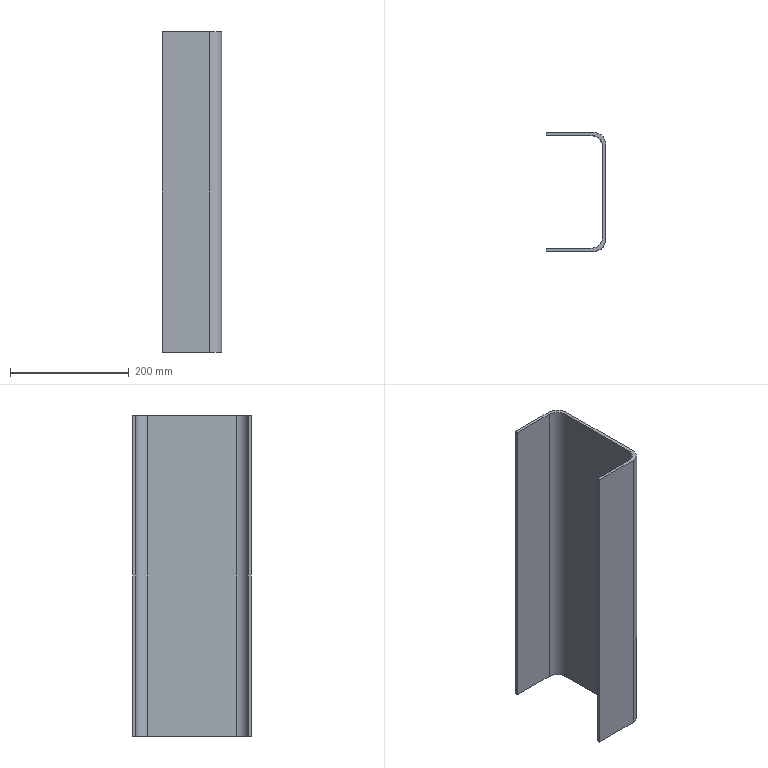Component | NX | PERFIL_U | 1 solid | 14 faces | box 100 x 200 x 540 mm | volume 1053000 mm3 | plane 10 | cylinder 4 | commonest cylinder face diameters 40 x4
STEP:
#1=CARTESIAN_POINT('',(0.,0.,0.));
#2=DIRECTION('',(0.,0.,1.));
#3=DIRECTION('',(1.,0.,0.));
#4=AXIS2_PLACEMENT_3D('',#1,#2,#3);
#5=CARTESIAN_POINT('',(0.,-234.8,700.));
#6=VERTEX_POINT('',#5);
#7=CARTESIAN_POINT('',(80.,-234.8,700.));
#8=VERTEX_POINT('',#7);
#9=CARTESIAN_POINT('',(0.,-234.8,700.));
#10=DIRECTION('',(1.,0.,0.));
#11=VECTOR('',#10,1.);
#12=LINE('',#9,#11);
#13=CARTESIAN_POINT('',(0.,-234.8,160.));
#14=DIRECTION('',(0.,-1.,0.));
#15=DIRECTION('',(1.,0.,0.));
#16=AXIS2_PLACEMENT_3D('',#13,#14,#15);
#17=PLANE('',#16);
#18=CARTESIAN_POINT('',(0.,540.));
#19=DIRECTION('',(1.,0.));
#20=VECTOR('',#19,1.);
#21=LINE('',#18,#20);
#22=(GEOMETRIC_REPRESENTATION_CONTEXT(2)PARAMETRIC_REPRESENTATION_CONTEXT()REPRESENTATION_CONTEXT('',''));
#23=DEFINITIONAL_REPRESENTATION('',(#21),#22);
#24=PCURVE('',#17,#23);
#25=CARTESIAN_POINT('',(100.,-234.8,700.));
#26=DIRECTION('',(0.,0.,-1.));
#27=DIRECTION('',(1.,0.,0.));
#28=AXIS2_PLACEMENT_3D('',#25,#26,#27);
#29=PLANE('',#28);
#30=CARTESIAN_POINT('',(-100.,0.));
#31=DIRECTION('',(1.,0.));
#32=VECTOR('',#31,1.);
#33=LINE('',#30,#32);
#34=(GEOMETRIC_REPRESENTATION_CONTEXT(2)PARAMETRIC_REPRESENTATION_CONTEXT()REPRESENTATION_CONTEXT('',''));
#35=DEFINITIONAL_REPRESENTATION('',(#33),#34);
#36=PCURVE('',#29,#35);
#37=SURFACE_CURVE('',#12,(#24,#36),.PCURVE_S1.);
#38=EDGE_CURVE('',#6,#8,#37,.T.);
#39=ORIENTED_EDGE('',*,*,#38,.T.);
#40=CARTESIAN_POINT('',(80.,-234.8,160.));
#41=VERTEX_POINT('',#40);
#42=CARTESIAN_POINT('',(80.,-234.8,160.));
#43=DIRECTION('',(0.,0.,-1.));
#44=VECTOR('',#43,1.);
#45=LINE('',#42,#44);
#46=CARTESIAN_POINT('',(80.,0.));
#47=DIRECTION('',(0.,-1.));
#48=VECTOR('',#47,1.);
#49=LINE('',#46,#48);
#50=(GEOMETRIC_REPRESENTATION_CONTEXT(2)PARAMETRIC_REPRESENTATION_CONTEXT()REPRESENTATION_CONTEXT('',''));
#51=DEFINITIONAL_REPRESENTATION('',(#49),#50);
#52=PCURVE('',#17,#51);
#53=CARTESIAN_POINT('',(80.,-254.8,160.));
#54=DIRECTION('',(0.,0.,1.));
#55=DIRECTION('',(-1.,0.,0.));
#56=AXIS2_PLACEMENT_3D('',#53,#54,#55);
#57=CYLINDRICAL_SURFACE('',#56,20.);
#58=CARTESIAN_POINT('',(4.712,0.));
#59=DIRECTION('',(0.,-1.));
#60=VECTOR('',#59,1.);
#61=LINE('',#58,#60);
#62=(GEOMETRIC_REPRESENTATION_CONTEXT(2)PARAMETRIC_REPRESENTATION_CONTEXT()REPRESENTATION_CONTEXT('',''));
#63=DEFINITIONAL_REPRESENTATION('',(#61),#62);
#64=PCURVE('',#57,#63);
#65=SURFACE_CURVE('',#45,(#52,#64),.PCURVE_S1.);
#66=EDGE_CURVE('',#8,#41,#65,.T.);
#67=ORIENTED_EDGE('',*,*,#66,.T.);
#68=CARTESIAN_POINT('',(0.,-234.8,160.));
#69=VERTEX_POINT('',#68);
#70=CARTESIAN_POINT('',(0.,-234.8,160.));
#71=DIRECTION('',(1.,0.,0.));
#72=VECTOR('',#71,1.);
#73=LINE('',#70,#72);
#74=CARTESIAN_POINT('',(0.,0.));
#75=DIRECTION('',(1.,0.));
#76=VECTOR('',#75,1.);
#77=LINE('',#74,#76);
#78=(GEOMETRIC_REPRESENTATION_CONTEXT(2)PARAMETRIC_REPRESENTATION_CONTEXT()REPRESENTATION_CONTEXT('',''));
#79=DEFINITIONAL_REPRESENTATION('',(#77),#78);
#80=PCURVE('',#17,#79);
#81=CARTESIAN_POINT('',(100.,-234.8,160.));
#82=DIRECTION('',(0.,0.,-1.));
#83=DIRECTION('',(1.,0.,0.));
#84=AXIS2_PLACEMENT_3D('',#81,#82,#83);
#85=PLANE('',#84);
#86=CARTESIAN_POINT('',(-100.,0.));
#87=DIRECTION('',(1.,0.));
#88=VECTOR('',#87,1.);
#89=LINE('',#86,#88);
#90=(GEOMETRIC_REPRESENTATION_CONTEXT(2)PARAMETRIC_REPRESENTATION_CONTEXT()REPRESENTATION_CONTEXT('',''));
#91=DEFINITIONAL_REPRESENTATION('',(#89),#90);
#92=PCURVE('',#85,#91);
#93=SURFACE_CURVE('',#73,(#80,#92),.PCURVE_S1.);
#94=EDGE_CURVE('',#69,#41,#93,.T.);
#95=ORIENTED_EDGE('',*,*,#94,.F.);
#96=CARTESIAN_POINT('',(0.,-234.8,160.));
#97=DIRECTION('',(0.,0.,1.));
#98=VECTOR('',#97,1.);
#99=LINE('',#96,#98);
#100=CARTESIAN_POINT('',(0.,0.));
#101=DIRECTION('',(0.,1.));
#102=VECTOR('',#101,1.);
#103=LINE('',#100,#102);
#104=(GEOMETRIC_REPRESENTATION_CONTEXT(2)PARAMETRIC_REPRESENTATION_CONTEXT()REPRESENTATION_CONTEXT('',''));
#105=DEFINITIONAL_REPRESENTATION('',(#103),#104);
#106=PCURVE('',#17,#105);
#107=CARTESIAN_POINT('',(0.,-239.8,160.));
#108=DIRECTION('',(1.,0.,0.));
#109=DIRECTION('',(0.,1.,0.));
#110=AXIS2_PLACEMENT_3D('',#107,#108,#109);
#111=PLANE('',#110);
#112=CARTESIAN_POINT('',(5.,0.));
#113=DIRECTION('',(0.,1.));
#114=VECTOR('',#113,1.);
#115=LINE('',#112,#114);
#116=(GEOMETRIC_REPRESENTATION_CONTEXT(2)PARAMETRIC_REPRESENTATION_CONTEXT()REPRESENTATION_CONTEXT('',''));
#117=DEFINITIONAL_REPRESENTATION('',(#115),#116);
#118=PCURVE('',#111,#117);
#119=SURFACE_CURVE('',#99,(#106,#118),.PCURVE_S1.);
#120=EDGE_CURVE('',#69,#6,#119,.T.);
#121=ORIENTED_EDGE('',*,*,#120,.T.);
#122=EDGE_LOOP('',(#39,#67,#95,#121));
#123=FACE_BOUND('',#122,.T.);
#124=ADVANCED_FACE('',(#123),#17,.F.);
#125=CARTESIAN_POINT('',(100.,-254.8,700.));
#126=VERTEX_POINT('',#125);
#127=CARTESIAN_POINT('',(100.,-414.8,700.));
#128=VERTEX_POINT('',#127);
#129=CARTESIAN_POINT('',(100.,-234.8,700.));
#130=DIRECTION('',(0.,-1.,0.));
#131=VECTOR('',#130,1.);
#132=LINE('',#129,#131);
#133=CARTESIAN_POINT('',(100.,-234.8,160.));
#134=DIRECTION('',(-1.,0.,0.));
#135=DIRECTION('',(0.,-1.,0.));
#136=AXIS2_PLACEMENT_3D('',#133,#134,#135);
#137=PLANE('',#136);
#138=CARTESIAN_POINT('',(0.,540.));
#139=DIRECTION('',(1.,0.));
#140=VECTOR('',#139,1.);
#141=LINE('',#138,#140);
#142=(GEOMETRIC_REPRESENTATION_CONTEXT(2)PARAMETRIC_REPRESENTATION_CONTEXT()REPRESENTATION_CONTEXT('',''));
#143=DEFINITIONAL_REPRESENTATION('',(#141),#142);
#144=PCURVE('',#137,#143);
#145=CARTESIAN_POINT('',(0.,0.));
#146=DIRECTION('',(0.,1.));
#147=VECTOR('',#146,1.);
#148=LINE('',#145,#147);
#149=(GEOMETRIC_REPRESENTATION_CONTEXT(2)PARAMETRIC_REPRESENTATION_CONTEXT()REPRESENTATION_CONTEXT('',''));
#150=DEFINITIONAL_REPRESENTATION('',(#148),#149);
#151=PCURVE('',#29,#150);
#152=SURFACE_CURVE('',#132,(#144,#151),.PCURVE_S1.);
#153=EDGE_CURVE('',#126,#128,#152,.T.);
#154=ORIENTED_EDGE('',*,*,#153,.T.);
#155=CARTESIAN_POINT('',(100.,-414.8,160.));
#156=VERTEX_POINT('',#155);
#157=CARTESIAN_POINT('',(100.,-414.8,160.));
#158=DIRECTION('',(0.,0.,-1.));
#159=VECTOR('',#158,1.);
#160=LINE('',#157,#159);
#161=CARTESIAN_POINT('',(180.,0.));
#162=DIRECTION('',(0.,-1.));
#163=VECTOR('',#162,1.);
#164=LINE('',#161,#163);
#165=(GEOMETRIC_REPRESENTATION_CONTEXT(2)PARAMETRIC_REPRESENTATION_CONTEXT()REPRESENTATION_CONTEXT('',''));
#166=DEFINITIONAL_REPRESENTATION('',(#164),#165);
#167=PCURVE('',#137,#166);
#168=CARTESIAN_POINT('',(80.,-414.8,160.));
#169=DIRECTION('',(0.,0.,1.));
#170=DIRECTION('',(-1.,0.,0.));
#171=AXIS2_PLACEMENT_3D('',#168,#169,#170);
#172=CYLINDRICAL_SURFACE('',#171,20.);
#173=CARTESIAN_POINT('',(3.142,0.));
#174=DIRECTION('',(0.,-1.));
#175=VECTOR('',#174,1.);
#176=LINE('',#173,#175);
#177=(GEOMETRIC_REPRESENTATION_CONTEXT(2)PARAMETRIC_REPRESENTATION_CONTEXT()REPRESENTATION_CONTEXT('',''));
#178=DEFINITIONAL_REPRESENTATION('',(#176),#177);
#179=PCURVE('',#172,#178);
#180=SURFACE_CURVE('',#160,(#167,#179),.PCURVE_S1.);
#181=EDGE_CURVE('',#128,#156,#180,.T.);
#182=ORIENTED_EDGE('',*,*,#181,.T.);
#183=CARTESIAN_POINT('',(100.,-254.8,160.));
#184=VERTEX_POINT('',#183);
#185=CARTESIAN_POINT('',(100.,-234.8,160.));
#186=DIRECTION('',(0.,-1.,0.));
#187=VECTOR('',#186,1.);
#188=LINE('',#185,#187);
#189=CARTESIAN_POINT('',(0.,0.));
#190=DIRECTION('',(1.,0.));
#191=VECTOR('',#190,1.);
#192=LINE('',#189,#191);
#193=(GEOMETRIC_REPRESENTATION_CONTEXT(2)PARAMETRIC_REPRESENTATION_CONTEXT()REPRESENTATION_CONTEXT('',''));
#194=DEFINITIONAL_REPRESENTATION('',(#192),#193);
#195=PCURVE('',#137,#194);
#196=CARTESIAN_POINT('',(0.,0.));
#197=DIRECTION('',(0.,1.));
#198=VECTOR('',#197,1.);
#199=LINE('',#196,#198);
#200=(GEOMETRIC_REPRESENTATION_CONTEXT(2)PARAMETRIC_REPRESENTATION_CONTEXT()REPRESENTATION_CONTEXT('',''));
#201=DEFINITIONAL_REPRESENTATION('',(#199),#200);
#202=PCURVE('',#85,#201);
#203=SURFACE_CURVE('',#188,(#195,#202),.PCURVE_S1.);
#204=EDGE_CURVE('',#184,#156,#203,.T.);
#205=ORIENTED_EDGE('',*,*,#204,.F.);
#206=CARTESIAN_POINT('',(100.,-254.8,160.));
#207=DIRECTION('',(0.,0.,1.));
#208=VECTOR('',#207,1.);
#209=LINE('',#206,#208);
#210=CARTESIAN_POINT('',(20.,0.));
#211=DIRECTION('',(0.,1.));
#212=VECTOR('',#211,1.);
#213=LINE('',#210,#212);
#214=(GEOMETRIC_REPRESENTATION_CONTEXT(2)PARAMETRIC_REPRESENTATION_CONTEXT()REPRESENTATION_CONTEXT('',''));
#215=DEFINITIONAL_REPRESENTATION('',(#213),#214);
#216=PCURVE('',#137,#215);
#217=CARTESIAN_POINT('',(3.142,0.));
#218=DIRECTION('',(0.,1.));
#219=VECTOR('',#218,1.);
#220=LINE('',#217,#219);
#221=(GEOMETRIC_REPRESENTATION_CONTEXT(2)PARAMETRIC_REPRESENTATION_CONTEXT()REPRESENTATION_CONTEXT('',''));
#222=DEFINITIONAL_REPRESENTATION('',(#220),#221);
#223=PCURVE('',#57,#222);
#224=SURFACE_CURVE('',#209,(#216,#223),.PCURVE_S1.);
#225=EDGE_CURVE('',#184,#126,#224,.T.);
#226=ORIENTED_EDGE('',*,*,#225,.T.);
#227=EDGE_LOOP('',(#154,#182,#205,#226));
#228=FACE_BOUND('',#227,.T.);
#229=ADVANCED_FACE('',(#228),#137,.F.);
#230=CARTESIAN_POINT('',(80.,-434.8,160.));
#231=VERTEX_POINT('',#230);
#232=CARTESIAN_POINT('',(0.,-434.8,160.));
#233=VERTEX_POINT('',#232);
#234=CARTESIAN_POINT('',(100.,-434.8,160.));
#235=DIRECTION('',(-1.,0.,0.));
#236=VECTOR('',#235,1.);
#237=LINE('',#234,#236);
#238=CARTESIAN_POINT('',(100.,-434.8,160.));
#239=DIRECTION('',(0.,1.,0.));
#240=DIRECTION('',(-1.,0.,0.));
#241=AXIS2_PLACEMENT_3D('',#238,#239,#240);
#242=PLANE('',#241);
#243=CARTESIAN_POINT('',(0.,0.));
#244=DIRECTION('',(1.,0.));
#245=VECTOR('',#244,1.);
#246=LINE('',#243,#245);
#247=(GEOMETRIC_REPRESENTATION_CONTEXT(2)PARAMETRIC_REPRESENTATION_CONTEXT()REPRESENTATION_CONTEXT('',''));
#248=DEFINITIONAL_REPRESENTATION('',(#246),#247);
#249=PCURVE('',#242,#248);
#250=CARTESIAN_POINT('',(0.,200.));
#251=DIRECTION('',(-1.,0.));
#252=VECTOR('',#251,1.);
#253=LINE('',#250,#252);
#254=(GEOMETRIC_REPRESENTATION_CONTEXT(2)PARAMETRIC_REPRESENTATION_CONTEXT()REPRESENTATION_CONTEXT('',''));
#255=DEFINITIONAL_REPRESENTATION('',(#253),#254);
#256=PCURVE('',#85,#255);
#257=SURFACE_CURVE('',#237,(#249,#256),.PCURVE_S1.);
#258=EDGE_CURVE('',#231,#233,#257,.T.);
#259=ORIENTED_EDGE('',*,*,#258,.F.);
#260=CARTESIAN_POINT('',(80.,-434.8,700.));
#261=VERTEX_POINT('',#260);
#262=CARTESIAN_POINT('',(80.,-434.8,160.));
#263=DIRECTION('',(0.,0.,1.));
#264=VECTOR('',#263,1.);
#265=LINE('',#262,#264);
#266=CARTESIAN_POINT('',(20.,0.));
#267=DIRECTION('',(0.,1.));
#268=VECTOR('',#267,1.);
#269=LINE('',#266,#268);
#270=(GEOMETRIC_REPRESENTATION_CONTEXT(2)PARAMETRIC_REPRESENTATION_CONTEXT()REPRESENTATION_CONTEXT('',''));
#271=DEFINITIONAL_REPRESENTATION('',(#269),#270);
#272=PCURVE('',#242,#271);
#273=CARTESIAN_POINT('',(1.571,0.));
#274=DIRECTION('',(0.,1.));
#275=VECTOR('',#274,1.);
#276=LINE('',#273,#275);
#277=(GEOMETRIC_REPRESENTATION_CONTEXT(2)PARAMETRIC_REPRESENTATION_CONTEXT()REPRESENTATION_CONTEXT('',''));
#278=DEFINITIONAL_REPRESENTATION('',(#276),#277);
#279=PCURVE('',#172,#278);
#280=SURFACE_CURVE('',#265,(#272,#279),.PCURVE_S1.);
#281=EDGE_CURVE('',#231,#261,#280,.T.);
#282=ORIENTED_EDGE('',*,*,#281,.T.);
#283=CARTESIAN_POINT('',(0.,-434.8,700.));
#284=VERTEX_POINT('',#283);
#285=CARTESIAN_POINT('',(100.,-434.8,700.));
#286=DIRECTION('',(-1.,0.,0.));
#287=VECTOR('',#286,1.);
#288=LINE('',#285,#287);
#289=CARTESIAN_POINT('',(0.,540.));
#290=DIRECTION('',(1.,0.));
#291=VECTOR('',#290,1.);
#292=LINE('',#289,#291);
#293=(GEOMETRIC_REPRESENTATION_CONTEXT(2)PARAMETRIC_REPRESENTATION_CONTEXT()REPRESENTATION_CONTEXT('',''));
#294=DEFINITIONAL_REPRESENTATION('',(#292),#293);
#295=PCURVE('',#242,#294);
#296=CARTESIAN_POINT('',(0.,200.));
#297=DIRECTION('',(-1.,0.));
#298=VECTOR('',#297,1.);
#299=LINE('',#296,#298);
#300=(GEOMETRIC_REPRESENTATION_CONTEXT(2)PARAMETRIC_REPRESENTATION_CONTEXT()REPRESENTATION_CONTEXT('',''));
#301=DEFINITIONAL_REPRESENTATION('',(#299),#300);
#302=PCURVE('',#29,#301);
#303=SURFACE_CURVE('',#288,(#295,#302),.PCURVE_S1.);
#304=EDGE_CURVE('',#261,#284,#303,.T.);
#305=ORIENTED_EDGE('',*,*,#304,.T.);
#306=CARTESIAN_POINT('',(0.,-434.8,160.));
#307=DIRECTION('',(0.,0.,1.));
#308=VECTOR('',#307,1.);
#309=LINE('',#306,#308);
#310=CARTESIAN_POINT('',(100.,0.));
#311=DIRECTION('',(0.,1.));
#312=VECTOR('',#311,1.);
#313=LINE('',#310,#312);
#314=(GEOMETRIC_REPRESENTATION_CONTEXT(2)PARAMETRIC_REPRESENTATION_CONTEXT()REPRESENTATION_CONTEXT('',''));
#315=DEFINITIONAL_REPRESENTATION('',(#313),#314);
#316=PCURVE('',#242,#315);
#317=CARTESIAN_POINT('',(0.,-434.8,160.));
#318=DIRECTION('',(1.,0.,0.));
#319=DIRECTION('',(0.,1.,0.));
#320=AXIS2_PLACEMENT_3D('',#317,#318,#319);
#321=PLANE('',#320);
#322=CARTESIAN_POINT('',(0.,0.));
#323=DIRECTION('',(0.,1.));
#324=VECTOR('',#323,1.);
#325=LINE('',#322,#324);
#326=(GEOMETRIC_REPRESENTATION_CONTEXT(2)PARAMETRIC_REPRESENTATION_CONTEXT()REPRESENTATION_CONTEXT('',''));
#327=DEFINITIONAL_REPRESENTATION('',(#325),#326);
#328=PCURVE('',#321,#327);
#329=SURFACE_CURVE('',#309,(#316,#328),.PCURVE_S1.);
#330=EDGE_CURVE('',#233,#284,#329,.T.);
#331=ORIENTED_EDGE('',*,*,#330,.F.);
#332=EDGE_LOOP('',(#259,#282,#305,#331));
#333=FACE_BOUND('',#332,.T.);
#334=ADVANCED_FACE('',(#333),#242,.F.);
#335=CARTESIAN_POINT('',(0.,-429.8,700.));
#336=VERTEX_POINT('',#335);
#337=CARTESIAN_POINT('',(0.,-434.8,700.));
#338=DIRECTION('',(0.,1.,0.));
#339=VECTOR('',#338,1.);
#340=LINE('',#337,#339);
#341=CARTESIAN_POINT('',(0.,540.));
#342=DIRECTION('',(1.,0.));
#343=VECTOR('',#342,1.);
#344=LINE('',#341,#343);
#345=(GEOMETRIC_REPRESENTATION_CONTEXT(2)PARAMETRIC_REPRESENTATION_CONTEXT()REPRESENTATION_CONTEXT('',''));
#346=DEFINITIONAL_REPRESENTATION('',(#344),#345);
#347=PCURVE('',#321,#346);
#348=CARTESIAN_POINT('',(-100.,200.));
#349=DIRECTION('',(0.,-1.));
#350=VECTOR('',#349,1.);
#351=LINE('',#348,#350);
#352=(GEOMETRIC_REPRESENTATION_CONTEXT(2)PARAMETRIC_REPRESENTATION_CONTEXT()REPRESENTATION_CONTEXT('',''));
#353=DEFINITIONAL_REPRESENTATION('',(#351),#352);
#354=PCURVE('',#29,#353);
#355=SURFACE_CURVE('',#340,(#347,#354),.PCURVE_S1.);
#356=EDGE_CURVE('',#284,#336,#355,.T.);
#357=ORIENTED_EDGE('',*,*,#356,.T.);
#358=CARTESIAN_POINT('',(0.,-429.8,160.));
#359=VERTEX_POINT('',#358);
#360=CARTESIAN_POINT('',(0.,-429.8,160.));
#361=DIRECTION('',(0.,0.,1.));
#362=VECTOR('',#361,1.);
#363=LINE('',#360,#362);
#364=CARTESIAN_POINT('',(5.,0.));
#365=DIRECTION('',(0.,1.));
#366=VECTOR('',#365,1.);
#367=LINE('',#364,#366);
#368=(GEOMETRIC_REPRESENTATION_CONTEXT(2)PARAMETRIC_REPRESENTATION_CONTEXT()REPRESENTATION_CONTEXT('',''));
#369=DEFINITIONAL_REPRESENTATION('',(#367),#368);
#370=PCURVE('',#321,#369);
#371=CARTESIAN_POINT('',(0.,-429.8,160.));
#372=DIRECTION('',(0.,-1.,0.));
#373=DIRECTION('',(1.,0.,0.));
#374=AXIS2_PLACEMENT_3D('',#371,#372,#373);
#375=PLANE('',#374);
#376=CARTESIAN_POINT('',(0.,0.));
#377=DIRECTION('',(0.,1.));
#378=VECTOR('',#377,1.);
#379=LINE('',#376,#378);
#380=(GEOMETRIC_REPRESENTATION_CONTEXT(2)PARAMETRIC_REPRESENTATION_CONTEXT()REPRESENTATION_CONTEXT('',''));
#381=DEFINITIONAL_REPRESENTATION('',(#379),#380);
#382=PCURVE('',#375,#381);
#383=SURFACE_CURVE('',#363,(#370,#382),.PCURVE_S1.);
#384=EDGE_CURVE('',#359,#336,#383,.T.);
#385=ORIENTED_EDGE('',*,*,#384,.F.);
#386=CARTESIAN_POINT('',(0.,-434.8,160.));
#387=DIRECTION('',(0.,1.,0.));
#388=VECTOR('',#387,1.);
#389=LINE('',#386,#388);
#390=CARTESIAN_POINT('',(0.,0.));
#391=DIRECTION('',(1.,0.));
#392=VECTOR('',#391,1.);
#393=LINE('',#390,#392);
#394=(GEOMETRIC_REPRESENTATION_CONTEXT(2)PARAMETRIC_REPRESENTATION_CONTEXT()REPRESENTATION_CONTEXT('',''));
#395=DEFINITIONAL_REPRESENTATION('',(#393),#394);
#396=PCURVE('',#321,#395);
#397=CARTESIAN_POINT('',(-100.,200.));
#398=DIRECTION('',(0.,-1.));
#399=VECTOR('',#398,1.);
#400=LINE('',#397,#399);
#401=(GEOMETRIC_REPRESENTATION_CONTEXT(2)PARAMETRIC_REPRESENTATION_CONTEXT()REPRESENTATION_CONTEXT('',''));
#402=DEFINITIONAL_REPRESENTATION('',(#400),#401);
#403=PCURVE('',#85,#402);
#404=SURFACE_CURVE('',#389,(#396,#403),.PCURVE_S1.);
#405=EDGE_CURVE('',#233,#359,#404,.T.);
#406=ORIENTED_EDGE('',*,*,#405,.F.);
#407=ORIENTED_EDGE('',*,*,#330,.T.);
#408=EDGE_LOOP('',(#357,#385,#406,#407));
#409=FACE_BOUND('',#408,.T.);
#410=ADVANCED_FACE('',(#409),#321,.F.);
#411=CARTESIAN_POINT('',(75.,-429.8,700.));
#412=VERTEX_POINT('',#411);
#413=CARTESIAN_POINT('',(0.,-429.8,700.));
#414=DIRECTION('',(1.,0.,0.));
#415=VECTOR('',#414,1.);
#416=LINE('',#413,#415);
#417=CARTESIAN_POINT('',(0.,540.));
#418=DIRECTION('',(1.,0.));
#419=VECTOR('',#418,1.);
#420=LINE('',#417,#419);
#421=(GEOMETRIC_REPRESENTATION_CONTEXT(2)PARAMETRIC_REPRESENTATION_CONTEXT()REPRESENTATION_CONTEXT('',''));
#422=DEFINITIONAL_REPRESENTATION('',(#420),#421);
#423=PCURVE('',#375,#422);
#424=CARTESIAN_POINT('',(-100.,195.));
#425=DIRECTION('',(1.,0.));
#426=VECTOR('',#425,1.);
#427=LINE('',#424,#426);
#428=(GEOMETRIC_REPRESENTATION_CONTEXT(2)PARAMETRIC_REPRESENTATION_CONTEXT()REPRESENTATION_CONTEXT('',''));
#429=DEFINITIONAL_REPRESENTATION('',(#427),#428);
#430=PCURVE('',#29,#429);
#431=SURFACE_CURVE('',#416,(#423,#430),.PCURVE_S1.);
#432=EDGE_CURVE('',#336,#412,#431,.T.);
#433=ORIENTED_EDGE('',*,*,#432,.T.);
#434=CARTESIAN_POINT('',(75.,-429.8,160.));
#435=VERTEX_POINT('',#434);
#436=CARTESIAN_POINT('',(75.,-429.8,160.));
#437=DIRECTION('',(0.,0.,-1.));
#438=VECTOR('',#437,1.);
#439=LINE('',#436,#438);
#440=CARTESIAN_POINT('',(75.,0.));
#441=DIRECTION('',(0.,-1.));
#442=VECTOR('',#441,1.);
#443=LINE('',#440,#442);
#444=(GEOMETRIC_REPRESENTATION_CONTEXT(2)PARAMETRIC_REPRESENTATION_CONTEXT()REPRESENTATION_CONTEXT('',''));
#445=DEFINITIONAL_REPRESENTATION('',(#443),#444);
#446=PCURVE('',#375,#445);
#447=CARTESIAN_POINT('',(75.,-409.8,160.));
#448=DIRECTION('',(0.,0.,-1.));
#449=DIRECTION('',(1.,0.,0.));
#450=AXIS2_PLACEMENT_3D('',#447,#448,#449);
#451=CYLINDRICAL_SURFACE('',#450,20.);
#452=CARTESIAN_POINT('',(1.571,0.));
#453=DIRECTION('',(0.,1.));
#454=VECTOR('',#453,1.);
#455=LINE('',#452,#454);
#456=(GEOMETRIC_REPRESENTATION_CONTEXT(2)PARAMETRIC_REPRESENTATION_CONTEXT()REPRESENTATION_CONTEXT('',''));
#457=DEFINITIONAL_REPRESENTATION('',(#455),#456);
#458=PCURVE('',#451,#457);
#459=SURFACE_CURVE('',#439,(#446,#458),.PCURVE_S1.);
#460=EDGE_CURVE('',#412,#435,#459,.T.);
#461=ORIENTED_EDGE('',*,*,#460,.T.);
#462=CARTESIAN_POINT('',(0.,-429.8,160.));
#463=DIRECTION('',(1.,0.,0.));
#464=VECTOR('',#463,1.);
#465=LINE('',#462,#464);
#466=CARTESIAN_POINT('',(0.,0.));
#467=DIRECTION('',(1.,0.));
#468=VECTOR('',#467,1.);
#469=LINE('',#466,#468);
#470=(GEOMETRIC_REPRESENTATION_CONTEXT(2)PARAMETRIC_REPRESENTATION_CONTEXT()REPRESENTATION_CONTEXT('',''));
#471=DEFINITIONAL_REPRESENTATION('',(#469),#470);
#472=PCURVE('',#375,#471);
#473=CARTESIAN_POINT('',(-100.,195.));
#474=DIRECTION('',(1.,0.));
#475=VECTOR('',#474,1.);
#476=LINE('',#473,#475);
#477=(GEOMETRIC_REPRESENTATION_CONTEXT(2)PARAMETRIC_REPRESENTATION_CONTEXT()REPRESENTATION_CONTEXT('',''));
#478=DEFINITIONAL_REPRESENTATION('',(#476),#477);
#479=PCURVE('',#85,#478);
#480=SURFACE_CURVE('',#465,(#472,#479),.PCURVE_S1.);
#481=EDGE_CURVE('',#359,#435,#480,.T.);
#482=ORIENTED_EDGE('',*,*,#481,.F.);
#483=ORIENTED_EDGE('',*,*,#384,.T.);
#484=EDGE_LOOP('',(#433,#461,#482,#483));
#485=FACE_BOUND('',#484,.T.);
#486=ADVANCED_FACE('',(#485),#375,.F.);
#487=CARTESIAN_POINT('',(95.,-409.8,160.));
#488=VERTEX_POINT('',#487);
#489=CARTESIAN_POINT('',(95.,-259.8,160.));
#490=VERTEX_POINT('',#489);
#491=CARTESIAN_POINT('',(95.,-429.8,160.));
#492=DIRECTION('',(0.,1.,0.));
#493=VECTOR('',#492,1.);
#494=LINE('',#491,#493);
#495=CARTESIAN_POINT('',(95.,-429.8,160.));
#496=DIRECTION('',(1.,0.,0.));
#497=DIRECTION('',(0.,1.,0.));
#498=AXIS2_PLACEMENT_3D('',#495,#496,#497);
#499=PLANE('',#498);
#500=CARTESIAN_POINT('',(0.,0.));
#501=DIRECTION('',(1.,0.));
#502=VECTOR('',#501,1.);
#503=LINE('',#500,#502);
#504=(GEOMETRIC_REPRESENTATION_CONTEXT(2)PARAMETRIC_REPRESENTATION_CONTEXT()REPRESENTATION_CONTEXT('',''));
#505=DEFINITIONAL_REPRESENTATION('',(#503),#504);
#506=PCURVE('',#499,#505);
#507=CARTESIAN_POINT('',(-5.,195.));
#508=DIRECTION('',(0.,-1.));
#509=VECTOR('',#508,1.);
#510=LINE('',#507,#509);
#511=(GEOMETRIC_REPRESENTATION_CONTEXT(2)PARAMETRIC_REPRESENTATION_CONTEXT()REPRESENTATION_CONTEXT('',''));
#512=DEFINITIONAL_REPRESENTATION('',(#510),#511);
#513=PCURVE('',#85,#512);
#514=SURFACE_CURVE('',#494,(#506,#513),.PCURVE_S1.);
#515=EDGE_CURVE('',#488,#490,#514,.T.);
#516=ORIENTED_EDGE('',*,*,#515,.F.);
#517=CARTESIAN_POINT('',(95.,-409.8,700.));
#518=VERTEX_POINT('',#517);
#519=CARTESIAN_POINT('',(95.,-409.8,700.));
#520=DIRECTION('',(0.,0.,1.));
#521=VECTOR('',#520,1.);
#522=LINE('',#519,#521);
#523=CARTESIAN_POINT('',(20.,540.));
#524=DIRECTION('',(0.,1.));
#525=VECTOR('',#524,1.);
#526=LINE('',#523,#525);
#527=(GEOMETRIC_REPRESENTATION_CONTEXT(2)PARAMETRIC_REPRESENTATION_CONTEXT()REPRESENTATION_CONTEXT('',''));
#528=DEFINITIONAL_REPRESENTATION('',(#526),#527);
#529=PCURVE('',#499,#528);
#530=CARTESIAN_POINT('',(0.,-540.));
#531=DIRECTION('',(0.,-1.));
#532=VECTOR('',#531,1.);
#533=LINE('',#530,#532);
#534=(GEOMETRIC_REPRESENTATION_CONTEXT(2)PARAMETRIC_REPRESENTATION_CONTEXT()REPRESENTATION_CONTEXT('',''));
#535=DEFINITIONAL_REPRESENTATION('',(#533),#534);
#536=PCURVE('',#451,#535);
#537=SURFACE_CURVE('',#522,(#529,#536),.PCURVE_S1.);
#538=EDGE_CURVE('',#488,#518,#537,.T.);
#539=ORIENTED_EDGE('',*,*,#538,.T.);
#540=CARTESIAN_POINT('',(95.,-259.8,700.));
#541=VERTEX_POINT('',#540);
#542=CARTESIAN_POINT('',(95.,-429.8,700.));
#543=DIRECTION('',(0.,1.,0.));
#544=VECTOR('',#543,1.);
#545=LINE('',#542,#544);
#546=CARTESIAN_POINT('',(0.,540.));
#547=DIRECTION('',(1.,0.));
#548=VECTOR('',#547,1.);
#549=LINE('',#546,#548);
#550=(GEOMETRIC_REPRESENTATION_CONTEXT(2)PARAMETRIC_REPRESENTATION_CONTEXT()REPRESENTATION_CONTEXT('',''));
#551=DEFINITIONAL_REPRESENTATION('',(#549),#550);
#552=PCURVE('',#499,#551);
#553=CARTESIAN_POINT('',(-5.,195.));
#554=DIRECTION('',(0.,-1.));
#555=VECTOR('',#554,1.);
#556=LINE('',#553,#555);
#557=(GEOMETRIC_REPRESENTATION_CONTEXT(2)PARAMETRIC_REPRESENTATION_CONTEXT()REPRESENTATION_CONTEXT('',''));
#558=DEFINITIONAL_REPRESENTATION('',(#556),#557);
#559=PCURVE('',#29,#558);
#560=SURFACE_CURVE('',#545,(#552,#559),.PCURVE_S1.);
#561=EDGE_CURVE('',#518,#541,#560,.T.);
#562=ORIENTED_EDGE('',*,*,#561,.T.);
#563=CARTESIAN_POINT('',(95.,-259.8,160.));
#564=DIRECTION('',(0.,0.,-1.));
#565=VECTOR('',#564,1.);
#566=LINE('',#563,#565);
#567=CARTESIAN_POINT('',(170.,0.));
#568=DIRECTION('',(0.,-1.));
#569=VECTOR('',#568,1.);
#570=LINE('',#567,#569);
#571=(GEOMETRIC_REPRESENTATION_CONTEXT(2)PARAMETRIC_REPRESENTATION_CONTEXT()REPRESENTATION_CONTEXT('',''));
#572=DEFINITIONAL_REPRESENTATION('',(#570),#571);
#573=PCURVE('',#499,#572);
#574=CARTESIAN_POINT('',(75.,-259.8,160.));
#575=DIRECTION('',(0.,0.,-1.));
#576=DIRECTION('',(1.,0.,0.));
#577=AXIS2_PLACEMENT_3D('',#574,#575,#576);
#578=CYLINDRICAL_SURFACE('',#577,20.);
#579=CARTESIAN_POINT('',(6.283,0.));
#580=DIRECTION('',(0.,1.));
#581=VECTOR('',#580,1.);
#582=LINE('',#579,#581);
#583=(GEOMETRIC_REPRESENTATION_CONTEXT(2)PARAMETRIC_REPRESENTATION_CONTEXT()REPRESENTATION_CONTEXT('',''));
#584=DEFINITIONAL_REPRESENTATION('',(#582),#583);
#585=PCURVE('',#578,#584);
#586=SURFACE_CURVE('',#566,(#573,#585),.PCURVE_S1.);
#587=EDGE_CURVE('',#541,#490,#586,.T.);
#588=ORIENTED_EDGE('',*,*,#587,.T.);
#589=EDGE_LOOP('',(#516,#539,#562,#588));
#590=FACE_BOUND('',#589,.T.);
#591=ADVANCED_FACE('',(#590),#499,.F.);
#592=CARTESIAN_POINT('',(75.,-239.8,160.));
#593=VERTEX_POINT('',#592);
#594=CARTESIAN_POINT('',(0.,-239.8,160.));
#595=VERTEX_POINT('',#594);
#596=CARTESIAN_POINT('',(95.,-239.8,160.));
#597=DIRECTION('',(-1.,0.,0.));
#598=VECTOR('',#597,1.);
#599=LINE('',#596,#598);
#600=CARTESIAN_POINT('',(95.,-239.8,160.));
#601=DIRECTION('',(0.,1.,0.));
#602=DIRECTION('',(-1.,0.,0.));
#603=AXIS2_PLACEMENT_3D('',#600,#601,#602);
#604=PLANE('',#603);
#605=CARTESIAN_POINT('',(0.,0.));
#606=DIRECTION('',(1.,0.));
#607=VECTOR('',#606,1.);
#608=LINE('',#605,#607);
#609=(GEOMETRIC_REPRESENTATION_CONTEXT(2)PARAMETRIC_REPRESENTATION_CONTEXT()REPRESENTATION_CONTEXT('',''));
#610=DEFINITIONAL_REPRESENTATION('',(#608),#609);
#611=PCURVE('',#604,#610);
#612=CARTESIAN_POINT('',(-5.,5.));
#613=DIRECTION('',(-1.,0.));
#614=VECTOR('',#613,1.);
#615=LINE('',#612,#614);
#616=(GEOMETRIC_REPRESENTATION_CONTEXT(2)PARAMETRIC_REPRESENTATION_CONTEXT()REPRESENTATION_CONTEXT('',''));
#617=DEFINITIONAL_REPRESENTATION('',(#615),#616);
#618=PCURVE('',#85,#617);
#619=SURFACE_CURVE('',#599,(#611,#618),.PCURVE_S1.);
#620=EDGE_CURVE('',#593,#595,#619,.T.);
#621=ORIENTED_EDGE('',*,*,#620,.F.);
#622=CARTESIAN_POINT('',(75.,-239.8,700.));
#623=VERTEX_POINT('',#622);
#624=CARTESIAN_POINT('',(75.,-239.8,700.));
#625=DIRECTION('',(0.,0.,1.));
#626=VECTOR('',#625,1.);
#627=LINE('',#624,#626);
#628=CARTESIAN_POINT('',(20.,540.));
#629=DIRECTION('',(0.,1.));
#630=VECTOR('',#629,1.);
#631=LINE('',#628,#630);
#632=(GEOMETRIC_REPRESENTATION_CONTEXT(2)PARAMETRIC_REPRESENTATION_CONTEXT()REPRESENTATION_CONTEXT('',''));
#633=DEFINITIONAL_REPRESENTATION('',(#631),#632);
#634=PCURVE('',#604,#633);
#635=CARTESIAN_POINT('',(4.712,-540.));
#636=DIRECTION('',(0.,-1.));
#637=VECTOR('',#636,1.);
#638=LINE('',#635,#637);
#639=(GEOMETRIC_REPRESENTATION_CONTEXT(2)PARAMETRIC_REPRESENTATION_CONTEXT()REPRESENTATION_CONTEXT('',''));
#640=DEFINITIONAL_REPRESENTATION('',(#638),#639);
#641=PCURVE('',#578,#640);
#642=SURFACE_CURVE('',#627,(#634,#641),.PCURVE_S1.);
#643=EDGE_CURVE('',#593,#623,#642,.T.);
#644=ORIENTED_EDGE('',*,*,#643,.T.);
#645=CARTESIAN_POINT('',(0.,-239.8,700.));
#646=VERTEX_POINT('',#645);
#647=CARTESIAN_POINT('',(95.,-239.8,700.));
#648=DIRECTION('',(-1.,0.,0.));
#649=VECTOR('',#648,1.);
#650=LINE('',#647,#649);
#651=CARTESIAN_POINT('',(0.,540.));
#652=DIRECTION('',(1.,0.));
#653=VECTOR('',#652,1.);
#654=LINE('',#651,#653);
#655=(GEOMETRIC_REPRESENTATION_CONTEXT(2)PARAMETRIC_REPRESENTATION_CONTEXT()REPRESENTATION_CONTEXT('',''));
#656=DEFINITIONAL_REPRESENTATION('',(#654),#655);
#657=PCURVE('',#604,#656);
#658=CARTESIAN_POINT('',(-5.,5.));
#659=DIRECTION('',(-1.,0.));
#660=VECTOR('',#659,1.);
#661=LINE('',#658,#660);
#662=(GEOMETRIC_REPRESENTATION_CONTEXT(2)PARAMETRIC_REPRESENTATION_CONTEXT()REPRESENTATION_CONTEXT('',''));
#663=DEFINITIONAL_REPRESENTATION('',(#661),#662);
#664=PCURVE('',#29,#663);
#665=SURFACE_CURVE('',#650,(#657,#664),.PCURVE_S1.);
#666=EDGE_CURVE('',#623,#646,#665,.T.);
#667=ORIENTED_EDGE('',*,*,#666,.T.);
#668=CARTESIAN_POINT('',(0.,-239.8,160.));
#669=DIRECTION('',(0.,0.,1.));
#670=VECTOR('',#669,1.);
#671=LINE('',#668,#670);
#672=CARTESIAN_POINT('',(95.,0.));
#673=DIRECTION('',(0.,1.));
#674=VECTOR('',#673,1.);
#675=LINE('',#672,#674);
#676=(GEOMETRIC_REPRESENTATION_CONTEXT(2)PARAMETRIC_REPRESENTATION_CONTEXT()REPRESENTATION_CONTEXT('',''));
#677=DEFINITIONAL_REPRESENTATION('',(#675),#676);
#678=PCURVE('',#604,#677);
#679=CARTESIAN_POINT('',(0.,0.));
#680=DIRECTION('',(0.,1.));
#681=VECTOR('',#680,1.);
#682=LINE('',#679,#681);
#683=(GEOMETRIC_REPRESENTATION_CONTEXT(2)PARAMETRIC_REPRESENTATION_CONTEXT()REPRESENTATION_CONTEXT('',''));
#684=DEFINITIONAL_REPRESENTATION('',(#682),#683);
#685=PCURVE('',#111,#684);
#686=SURFACE_CURVE('',#671,(#678,#685),.PCURVE_S1.);
#687=EDGE_CURVE('',#595,#646,#686,.T.);
#688=ORIENTED_EDGE('',*,*,#687,.F.);
#689=EDGE_LOOP('',(#621,#644,#667,#688));
#690=FACE_BOUND('',#689,.T.);
#691=ADVANCED_FACE('',(#690),#604,.F.);
#692=CARTESIAN_POINT('',(0.,-239.8,700.));
#693=DIRECTION('',(0.,1.,0.));
#694=VECTOR('',#693,1.);
#695=LINE('',#692,#694);
#696=CARTESIAN_POINT('',(0.,540.));
#697=DIRECTION('',(1.,0.));
#698=VECTOR('',#697,1.);
#699=LINE('',#696,#698);
#700=(GEOMETRIC_REPRESENTATION_CONTEXT(2)PARAMETRIC_REPRESENTATION_CONTEXT()REPRESENTATION_CONTEXT('',''));
#701=DEFINITIONAL_REPRESENTATION('',(#699),#700);
#702=PCURVE('',#111,#701);
#703=CARTESIAN_POINT('',(-100.,5.));
#704=DIRECTION('',(0.,-1.));
#705=VECTOR('',#704,1.);
#706=LINE('',#703,#705);
#707=(GEOMETRIC_REPRESENTATION_CONTEXT(2)PARAMETRIC_REPRESENTATION_CONTEXT()REPRESENTATION_CONTEXT('',''));
#708=DEFINITIONAL_REPRESENTATION('',(#706),#707);
#709=PCURVE('',#29,#708);
#710=SURFACE_CURVE('',#695,(#702,#709),.PCURVE_S1.);
#711=EDGE_CURVE('',#646,#6,#710,.T.);
#712=ORIENTED_EDGE('',*,*,#711,.T.);
#713=ORIENTED_EDGE('',*,*,#120,.F.);
#714=CARTESIAN_POINT('',(0.,-239.8,160.));
#715=DIRECTION('',(0.,1.,0.));
#716=VECTOR('',#715,1.);
#717=LINE('',#714,#716);
#718=CARTESIAN_POINT('',(0.,0.));
#719=DIRECTION('',(1.,0.));
#720=VECTOR('',#719,1.);
#721=LINE('',#718,#720);
#722=(GEOMETRIC_REPRESENTATION_CONTEXT(2)PARAMETRIC_REPRESENTATION_CONTEXT()REPRESENTATION_CONTEXT('',''));
#723=DEFINITIONAL_REPRESENTATION('',(#721),#722);
#724=PCURVE('',#111,#723);
#725=CARTESIAN_POINT('',(-100.,5.));
#726=DIRECTION('',(0.,-1.));
#727=VECTOR('',#726,1.);
#728=LINE('',#725,#727);
#729=(GEOMETRIC_REPRESENTATION_CONTEXT(2)PARAMETRIC_REPRESENTATION_CONTEXT()REPRESENTATION_CONTEXT('',''));
#730=DEFINITIONAL_REPRESENTATION('',(#728),#729);
#731=PCURVE('',#85,#730);
#732=SURFACE_CURVE('',#717,(#724,#731),.PCURVE_S1.);
#733=EDGE_CURVE('',#595,#69,#732,.T.);
#734=ORIENTED_EDGE('',*,*,#733,.F.);
#735=ORIENTED_EDGE('',*,*,#687,.T.);
#736=EDGE_LOOP('',(#712,#713,#734,#735));
#737=FACE_BOUND('',#736,.T.);
#738=ADVANCED_FACE('',(#737),#111,.F.);
#739=ORIENTED_EDGE('',*,*,#204,.T.);
#740=CARTESIAN_POINT('',(80.,-414.8,160.));
#741=DIRECTION('',(0.,0.,-1.));
#742=DIRECTION('',(1.,0.,0.));
#743=AXIS2_PLACEMENT_3D('',#740,#741,#742);
#744=CIRCLE('',#743,20.);
#745=CARTESIAN_POINT('',(-20.,180.));
#746=DIRECTION('',(1.,0.));
#747=AXIS2_PLACEMENT_2D('',#745,#746);
#748=CIRCLE('',#747,20.);
#749=(GEOMETRIC_REPRESENTATION_CONTEXT(2)PARAMETRIC_REPRESENTATION_CONTEXT()REPRESENTATION_CONTEXT('',''));
#750=DEFINITIONAL_REPRESENTATION('',(#748),#749);
#751=PCURVE('',#85,#750);
#752=CARTESIAN_POINT('',(3.142,0.));
#753=DIRECTION('',(-1.,0.));
#754=VECTOR('',#753,1.);
#755=LINE('',#752,#754);
#756=(GEOMETRIC_REPRESENTATION_CONTEXT(2)PARAMETRIC_REPRESENTATION_CONTEXT()REPRESENTATION_CONTEXT('',''));
#757=DEFINITIONAL_REPRESENTATION('',(#755),#756);
#758=PCURVE('',#172,#757);
#759=SURFACE_CURVE('',#744,(#751,#758),.PCURVE_S1.);
#760=EDGE_CURVE('',#156,#231,#759,.T.);
#761=ORIENTED_EDGE('',*,*,#760,.T.);
#762=ORIENTED_EDGE('',*,*,#258,.T.);
#763=ORIENTED_EDGE('',*,*,#405,.T.);
#764=ORIENTED_EDGE('',*,*,#481,.T.);
#765=CARTESIAN_POINT('',(75.,-409.8,160.));
#766=DIRECTION('',(0.,0.,1.));
#767=DIRECTION('',(1.,0.,0.));
#768=AXIS2_PLACEMENT_3D('',#765,#766,#767);
#769=CIRCLE('',#768,20.);
#770=CARTESIAN_POINT('',(-5.,175.));
#771=CARTESIAN_POINT('',(-5.,140.359));
#772=CARTESIAN_POINT('',(-35.,157.679));
#773=CARTESIAN_POINT('',(-65.,175.));
#774=CARTESIAN_POINT('',(-35.,192.321));
#775=CARTESIAN_POINT('',(-5.,209.641));
#776=CARTESIAN_POINT('',(-5.,175.));
#777=(BOUNDED_CURVE()B_SPLINE_CURVE(2,(#770,#771,#772,#773,#774,#775,#776),.UNSPECIFIED.,.T.,.F.)B_SPLINE_CURVE_WITH_KNOTS((1,2,2,2,2,1),(-2.094,0.,2.094,4.189,6.283,8.378),.UNSPECIFIED.)CURVE()GEOMETRIC_REPRESENTATION_ITEM()RATIONAL_B_SPLINE_CURVE((1.,0.5,1.,0.5,1.,0.5,1.))REPRESENTATION_ITEM(''));
#778=(GEOMETRIC_REPRESENTATION_CONTEXT(2)PARAMETRIC_REPRESENTATION_CONTEXT()REPRESENTATION_CONTEXT('',''));
#779=DEFINITIONAL_REPRESENTATION('',(#777),#778);
#780=PCURVE('',#85,#779);
#781=CARTESIAN_POINT('',(6.283,0.));
#782=DIRECTION('',(-1.,0.));
#783=VECTOR('',#782,1.);
#784=LINE('',#781,#783);
#785=(GEOMETRIC_REPRESENTATION_CONTEXT(2)PARAMETRIC_REPRESENTATION_CONTEXT()REPRESENTATION_CONTEXT('',''));
#786=DEFINITIONAL_REPRESENTATION('',(#784),#785);
#787=PCURVE('',#451,#786);
#788=SURFACE_CURVE('',#769,(#780,#787),.PCURVE_S1.);
#789=EDGE_CURVE('',#435,#488,#788,.T.);
#790=ORIENTED_EDGE('',*,*,#789,.T.);
#791=ORIENTED_EDGE('',*,*,#515,.T.);
#792=CARTESIAN_POINT('',(75.,-259.8,160.));
#793=DIRECTION('',(0.,0.,1.));
#794=DIRECTION('',(1.,0.,0.));
#795=AXIS2_PLACEMENT_3D('',#792,#793,#794);
#796=CIRCLE('',#795,20.);
#797=CARTESIAN_POINT('',(-5.,25.));
#798=CARTESIAN_POINT('',(-5.,-9.641));
#799=CARTESIAN_POINT('',(-35.,7.679));
#800=CARTESIAN_POINT('',(-65.,25.));
#801=CARTESIAN_POINT('',(-35.,42.321));
#802=CARTESIAN_POINT('',(-5.,59.641));
#803=CARTESIAN_POINT('',(-5.,25.));
#804=(BOUNDED_CURVE()B_SPLINE_CURVE(2,(#797,#798,#799,#800,#801,#802,#803),.UNSPECIFIED.,.T.,.F.)B_SPLINE_CURVE_WITH_KNOTS((1,2,2,2,2,1),(-2.094,0.,2.094,4.189,6.283,8.378),.UNSPECIFIED.)CURVE()GEOMETRIC_REPRESENTATION_ITEM()RATIONAL_B_SPLINE_CURVE((1.,0.5,1.,0.5,1.,0.5,1.))REPRESENTATION_ITEM(''));
#805=(GEOMETRIC_REPRESENTATION_CONTEXT(2)PARAMETRIC_REPRESENTATION_CONTEXT()REPRESENTATION_CONTEXT('',''));
#806=DEFINITIONAL_REPRESENTATION('',(#804),#805);
#807=PCURVE('',#85,#806);
#808=CARTESIAN_POINT('',(6.283,0.));
#809=DIRECTION('',(-1.,0.));
#810=VECTOR('',#809,1.);
#811=LINE('',#808,#810);
#812=(GEOMETRIC_REPRESENTATION_CONTEXT(2)PARAMETRIC_REPRESENTATION_CONTEXT()REPRESENTATION_CONTEXT('',''));
#813=DEFINITIONAL_REPRESENTATION('',(#811),#812);
#814=PCURVE('',#578,#813);
#815=SURFACE_CURVE('',#796,(#807,#814),.PCURVE_S1.);
#816=EDGE_CURVE('',#490,#593,#815,.T.);
#817=ORIENTED_EDGE('',*,*,#816,.T.);
#818=ORIENTED_EDGE('',*,*,#620,.T.);
#819=ORIENTED_EDGE('',*,*,#733,.T.);
#820=ORIENTED_EDGE('',*,*,#94,.T.);
#821=CARTESIAN_POINT('',(80.,-254.8,160.));
#822=DIRECTION('',(0.,0.,-1.));
#823=DIRECTION('',(1.,0.,0.));
#824=AXIS2_PLACEMENT_3D('',#821,#822,#823);
#825=CIRCLE('',#824,20.);
#826=CARTESIAN_POINT('',(-20.,20.));
#827=DIRECTION('',(1.,0.));
#828=AXIS2_PLACEMENT_2D('',#826,#827);
#829=CIRCLE('',#828,20.);
#830=(GEOMETRIC_REPRESENTATION_CONTEXT(2)PARAMETRIC_REPRESENTATION_CONTEXT()REPRESENTATION_CONTEXT('',''));
#831=DEFINITIONAL_REPRESENTATION('',(#829),#830);
#832=PCURVE('',#85,#831);
#833=CARTESIAN_POINT('',(9.425,0.));
#834=DIRECTION('',(-1.,0.));
#835=VECTOR('',#834,1.);
#836=LINE('',#833,#835);
#837=(GEOMETRIC_REPRESENTATION_CONTEXT(2)PARAMETRIC_REPRESENTATION_CONTEXT()REPRESENTATION_CONTEXT('',''));
#838=DEFINITIONAL_REPRESENTATION('',(#836),#837);
#839=PCURVE('',#57,#838);
#840=SURFACE_CURVE('',#825,(#832,#839),.PCURVE_S1.);
#841=EDGE_CURVE('',#41,#184,#840,.T.);
#842=ORIENTED_EDGE('',*,*,#841,.T.);
#843=EDGE_LOOP('',(#739,#761,#762,#763,#764,#790,#791,#817,#818,#819,#820,#842));
#844=FACE_BOUND('',#843,.T.);
#845=ADVANCED_FACE('',(#844),#85,.T.);
#846=ORIENTED_EDGE('',*,*,#304,.F.);
#847=CARTESIAN_POINT('',(80.,-414.8,700.));
#848=DIRECTION('',(0.,0.,1.));
#849=DIRECTION('',(1.,0.,0.));
#850=AXIS2_PLACEMENT_3D('',#847,#848,#849);
#851=CIRCLE('',#850,20.);
#852=CARTESIAN_POINT('',(0.,180.));
#853=CARTESIAN_POINT('',(0.,145.359));
#854=CARTESIAN_POINT('',(-30.,162.679));
#855=CARTESIAN_POINT('',(-60.,180.));
#856=CARTESIAN_POINT('',(-30.,197.321));
#857=CARTESIAN_POINT('',(0.,214.641));
#858=CARTESIAN_POINT('',(0.,180.));
#859=(BOUNDED_CURVE()B_SPLINE_CURVE(2,(#852,#853,#854,#855,#856,#857,#858),.UNSPECIFIED.,.T.,.F.)B_SPLINE_CURVE_WITH_KNOTS((1,2,2,2,2,1),(-2.094,0.,2.094,4.189,6.283,8.378),.UNSPECIFIED.)CURVE()GEOMETRIC_REPRESENTATION_ITEM()RATIONAL_B_SPLINE_CURVE((1.,0.5,1.,0.5,1.,0.5,1.))REPRESENTATION_ITEM(''));
#860=(GEOMETRIC_REPRESENTATION_CONTEXT(2)PARAMETRIC_REPRESENTATION_CONTEXT()REPRESENTATION_CONTEXT('',''));
#861=DEFINITIONAL_REPRESENTATION('',(#859),#860);
#862=PCURVE('',#29,#861);
#863=CARTESIAN_POINT('',(-3.142,540.));
#864=DIRECTION('',(1.,0.));
#865=VECTOR('',#864,1.);
#866=LINE('',#863,#865);
#867=(GEOMETRIC_REPRESENTATION_CONTEXT(2)PARAMETRIC_REPRESENTATION_CONTEXT()REPRESENTATION_CONTEXT('',''));
#868=DEFINITIONAL_REPRESENTATION('',(#866),#867);
#869=PCURVE('',#172,#868);
#870=SURFACE_CURVE('',#851,(#862,#869),.PCURVE_S1.);
#871=EDGE_CURVE('',#261,#128,#870,.T.);
#872=ORIENTED_EDGE('',*,*,#871,.T.);
#873=ORIENTED_EDGE('',*,*,#153,.F.);
#874=CARTESIAN_POINT('',(80.,-254.8,700.));
#875=DIRECTION('',(0.,0.,1.));
#876=DIRECTION('',(1.,0.,0.));
#877=AXIS2_PLACEMENT_3D('',#874,#875,#876);
#878=CIRCLE('',#877,20.);
#879=CARTESIAN_POINT('',(0.,20.));
#880=CARTESIAN_POINT('',(0.,-14.641));
#881=CARTESIAN_POINT('',(-30.,2.679));
#882=CARTESIAN_POINT('',(-60.,20.));
#883=CARTESIAN_POINT('',(-30.,37.321));
#884=CARTESIAN_POINT('',(0.,54.641));
#885=CARTESIAN_POINT('',(0.,20.));
#886=(BOUNDED_CURVE()B_SPLINE_CURVE(2,(#879,#880,#881,#882,#883,#884,#885),.UNSPECIFIED.,.T.,.F.)B_SPLINE_CURVE_WITH_KNOTS((1,2,2,2,2,1),(-2.094,0.,2.094,4.189,6.283,8.378),.UNSPECIFIED.)CURVE()GEOMETRIC_REPRESENTATION_ITEM()RATIONAL_B_SPLINE_CURVE((1.,0.5,1.,0.5,1.,0.5,1.))REPRESENTATION_ITEM(''));
#887=(GEOMETRIC_REPRESENTATION_CONTEXT(2)PARAMETRIC_REPRESENTATION_CONTEXT()REPRESENTATION_CONTEXT('',''));
#888=DEFINITIONAL_REPRESENTATION('',(#886),#887);
#889=PCURVE('',#29,#888);
#890=CARTESIAN_POINT('',(3.142,540.));
#891=DIRECTION('',(1.,0.));
#892=VECTOR('',#891,1.);
#893=LINE('',#890,#892);
#894=(GEOMETRIC_REPRESENTATION_CONTEXT(2)PARAMETRIC_REPRESENTATION_CONTEXT()REPRESENTATION_CONTEXT('',''));
#895=DEFINITIONAL_REPRESENTATION('',(#893),#894);
#896=PCURVE('',#57,#895);
#897=SURFACE_CURVE('',#878,(#889,#896),.PCURVE_S1.);
#898=EDGE_CURVE('',#126,#8,#897,.T.);
#899=ORIENTED_EDGE('',*,*,#898,.T.);
#900=ORIENTED_EDGE('',*,*,#38,.F.);
#901=ORIENTED_EDGE('',*,*,#711,.F.);
#902=ORIENTED_EDGE('',*,*,#666,.F.);
#903=CARTESIAN_POINT('',(75.,-259.8,700.));
#904=DIRECTION('',(0.,0.,-1.));
#905=DIRECTION('',(1.,0.,0.));
#906=AXIS2_PLACEMENT_3D('',#903,#904,#905);
#907=CIRCLE('',#906,20.);
#908=CARTESIAN_POINT('',(-25.,25.));
#909=DIRECTION('',(1.,0.));
#910=AXIS2_PLACEMENT_2D('',#908,#909);
#911=CIRCLE('',#910,20.);
#912=(GEOMETRIC_REPRESENTATION_CONTEXT(2)PARAMETRIC_REPRESENTATION_CONTEXT()REPRESENTATION_CONTEXT('',''));
#913=DEFINITIONAL_REPRESENTATION('',(#911),#912);
#914=PCURVE('',#29,#913);
#915=CARTESIAN_POINT('',(0.,-540.));
#916=DIRECTION('',(1.,0.));
#917=VECTOR('',#916,1.);
#918=LINE('',#915,#917);
#919=(GEOMETRIC_REPRESENTATION_CONTEXT(2)PARAMETRIC_REPRESENTATION_CONTEXT()REPRESENTATION_CONTEXT('',''));
#920=DEFINITIONAL_REPRESENTATION('',(#918),#919);
#921=PCURVE('',#578,#920);
#922=SURFACE_CURVE('',#907,(#914,#921),.PCURVE_S1.);
#923=EDGE_CURVE('',#623,#541,#922,.T.);
#924=ORIENTED_EDGE('',*,*,#923,.T.);
#925=ORIENTED_EDGE('',*,*,#561,.F.);
#926=CARTESIAN_POINT('',(75.,-409.8,700.));
#927=DIRECTION('',(0.,0.,-1.));
#928=DIRECTION('',(1.,0.,0.));
#929=AXIS2_PLACEMENT_3D('',#926,#927,#928);
#930=CIRCLE('',#929,20.);
#931=CARTESIAN_POINT('',(-25.,175.));
#932=DIRECTION('',(1.,0.));
#933=AXIS2_PLACEMENT_2D('',#931,#932);
#934=CIRCLE('',#933,20.);
#935=(GEOMETRIC_REPRESENTATION_CONTEXT(2)PARAMETRIC_REPRESENTATION_CONTEXT()REPRESENTATION_CONTEXT('',''));
#936=DEFINITIONAL_REPRESENTATION('',(#934),#935);
#937=PCURVE('',#29,#936);
#938=CARTESIAN_POINT('',(0.,-540.));
#939=DIRECTION('',(1.,0.));
#940=VECTOR('',#939,1.);
#941=LINE('',#938,#940);
#942=(GEOMETRIC_REPRESENTATION_CONTEXT(2)PARAMETRIC_REPRESENTATION_CONTEXT()REPRESENTATION_CONTEXT('',''));
#943=DEFINITIONAL_REPRESENTATION('',(#941),#942);
#944=PCURVE('',#451,#943);
#945=SURFACE_CURVE('',#930,(#937,#944),.PCURVE_S1.);
#946=EDGE_CURVE('',#518,#412,#945,.T.);
#947=ORIENTED_EDGE('',*,*,#946,.T.);
#948=ORIENTED_EDGE('',*,*,#432,.F.);
#949=ORIENTED_EDGE('',*,*,#356,.F.);
#950=EDGE_LOOP('',(#846,#872,#873,#899,#900,#901,#902,#924,#925,#947,#948,#949));
#951=FACE_BOUND('',#950,.T.);
#952=ADVANCED_FACE('',(#951),#29,.F.);
#953=ORIENTED_EDGE('',*,*,#760,.F.);
#954=ORIENTED_EDGE('',*,*,#181,.F.);
#955=ORIENTED_EDGE('',*,*,#871,.F.);
#956=ORIENTED_EDGE('',*,*,#281,.F.);
#957=EDGE_LOOP('',(#953,#954,#955,#956));
#958=FACE_BOUND('',#957,.T.);
#959=ADVANCED_FACE('',(#958),#172,.T.);
#960=ORIENTED_EDGE('',*,*,#841,.F.);
#961=ORIENTED_EDGE('',*,*,#66,.F.);
#962=ORIENTED_EDGE('',*,*,#898,.F.);
#963=ORIENTED_EDGE('',*,*,#225,.F.);
#964=EDGE_LOOP('',(#960,#961,#962,#963));
#965=FACE_BOUND('',#964,.T.);
#966=ADVANCED_FACE('',(#965),#57,.T.);
#967=ORIENTED_EDGE('',*,*,#538,.T.);
#968=ORIENTED_EDGE('',*,*,#946,.T.);
#969=ORIENTED_EDGE('',*,*,#460,.T.);
#970=ORIENTED_EDGE('',*,*,#789,.T.);
#971=EDGE_LOOP('',(#967,#968,#969,#970));
#972=FACE_BOUND('',#971,.F.);
#973=ADVANCED_FACE('',(#972),#451,.F.);
#974=ORIENTED_EDGE('',*,*,#643,.T.);
#975=ORIENTED_EDGE('',*,*,#923,.T.);
#976=ORIENTED_EDGE('',*,*,#587,.T.);
#977=ORIENTED_EDGE('',*,*,#816,.T.);
#978=EDGE_LOOP('',(#974,#975,#976,#977));
#979=FACE_BOUND('',#978,.F.);
#980=ADVANCED_FACE('',(#979),#578,.F.);
#981=CLOSED_SHELL('',(#124,#229,#334,#410,#486,#591,#691,#738,#845,#952,#959,#966,#973,#980));
#982=MANIFOLD_SOLID_BREP('',#981);
#983=(LENGTH_UNIT()NAMED_UNIT(*)SI_UNIT(.MILLI.,.METRE.));
#984=UNCERTAINTY_MEASURE_WITH_UNIT(LENGTH_MEASURE(0.0000001),#983,'','');
#985=(NAMED_UNIT(*)PLANE_ANGLE_UNIT()SI_UNIT($,.RADIAN.));
#986=(NAMED_UNIT(*)SI_UNIT($,.STERADIAN.)SOLID_ANGLE_UNIT());
#987=(GEOMETRIC_REPRESENTATION_CONTEXT(3)GLOBAL_UNCERTAINTY_ASSIGNED_CONTEXT((#984))GLOBAL_UNIT_ASSIGNED_CONTEXT((#983,#985,#986))REPRESENTATION_CONTEXT('',''));
#988=ADVANCED_BREP_SHAPE_REPRESENTATION('',(#4,#982),#987);